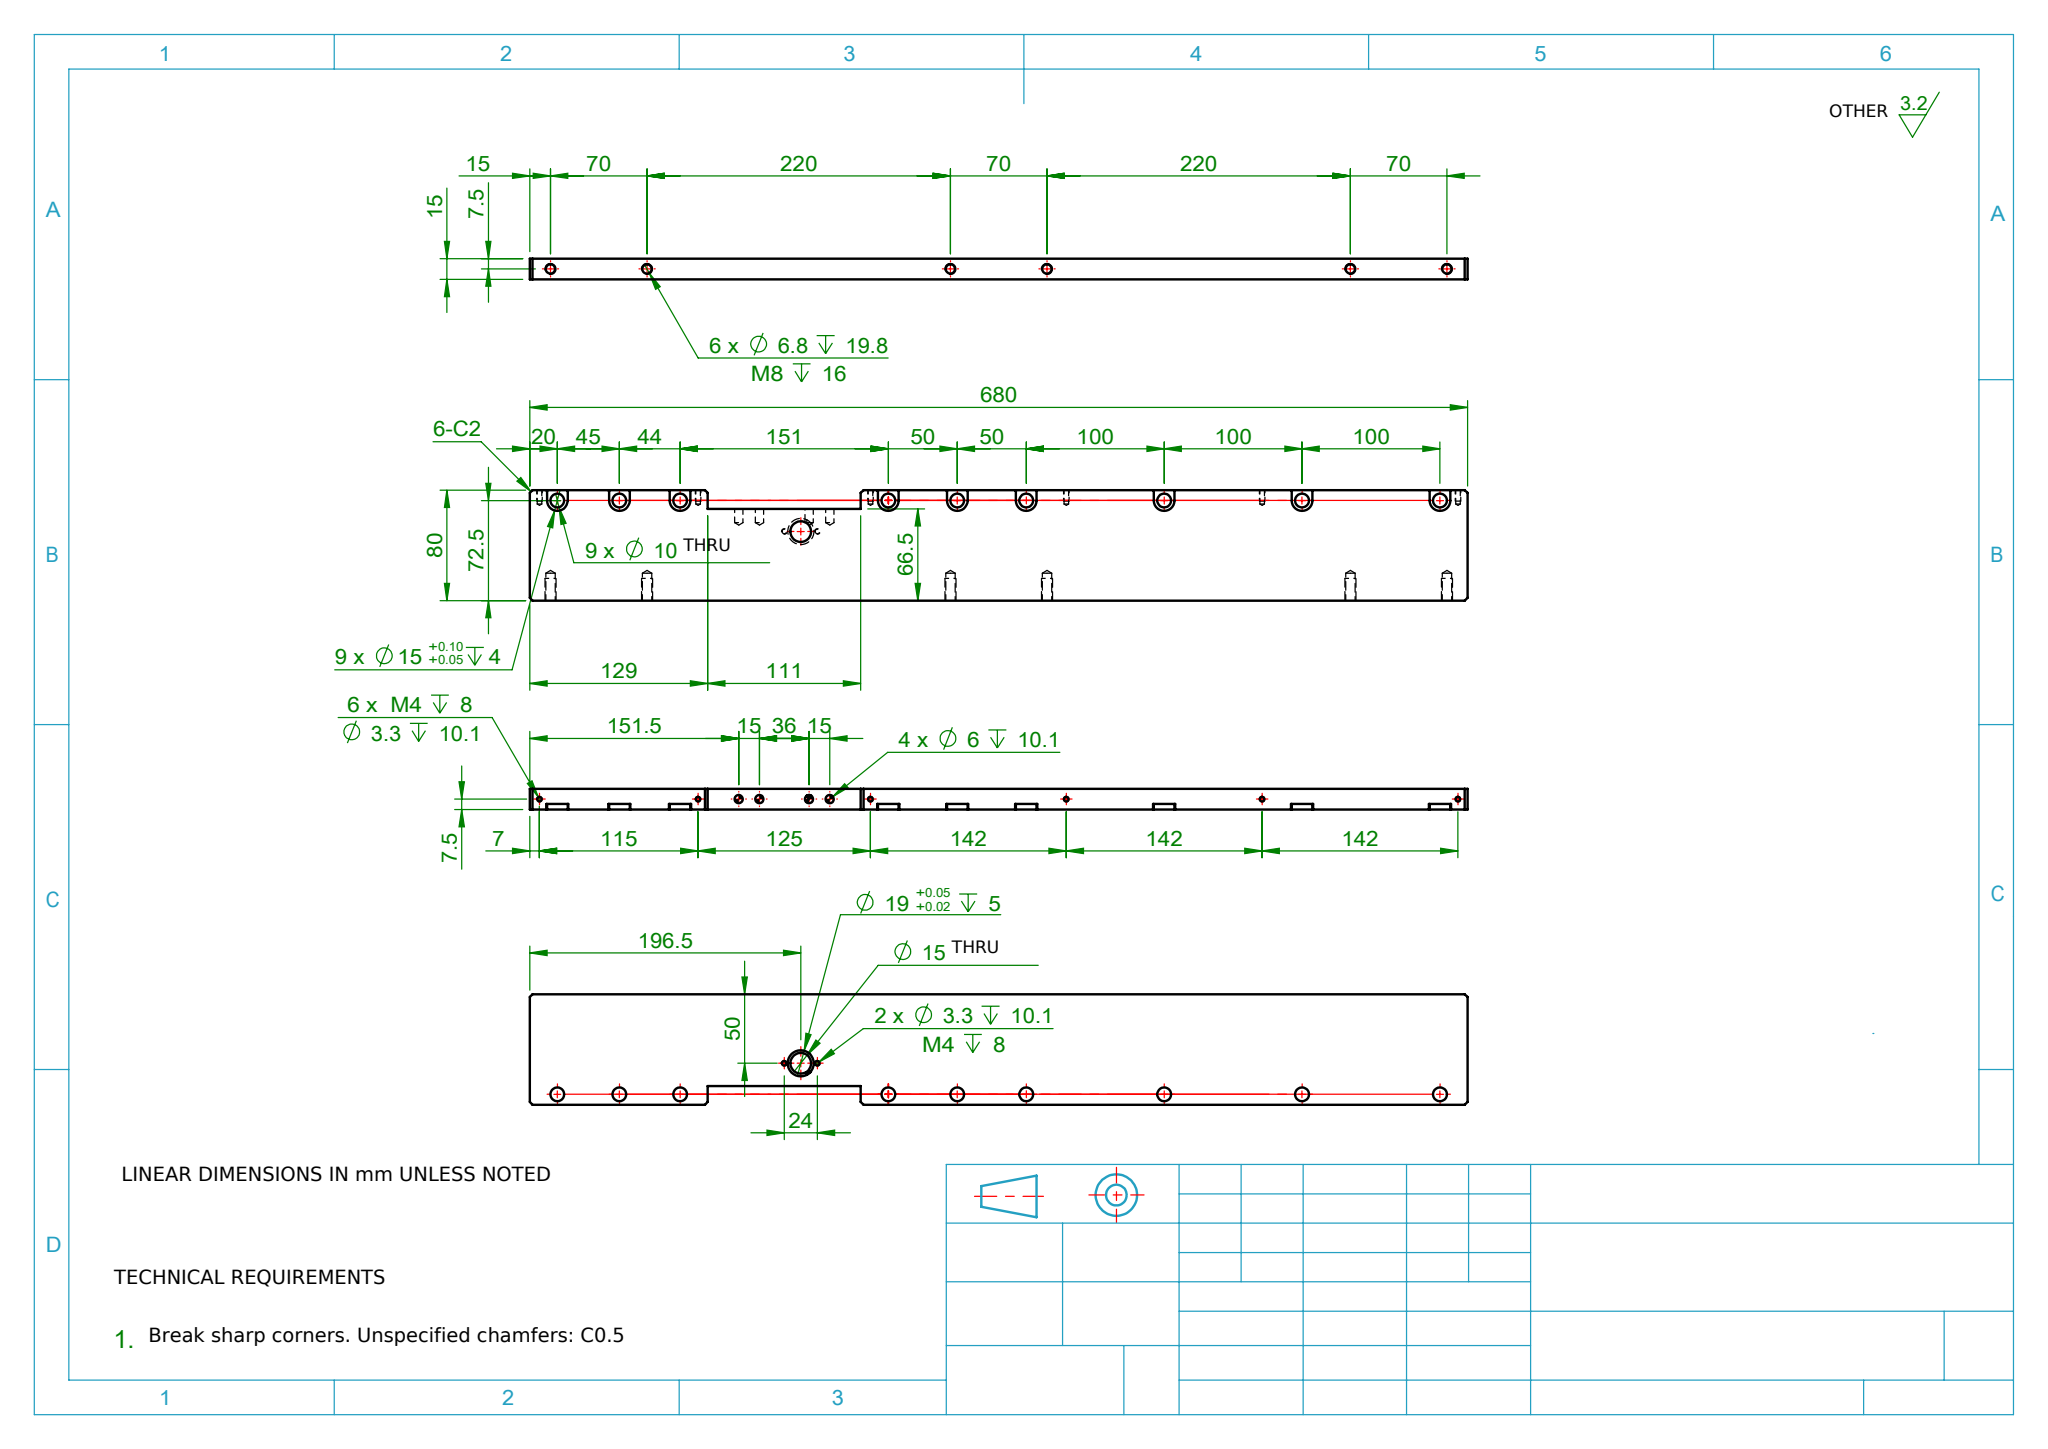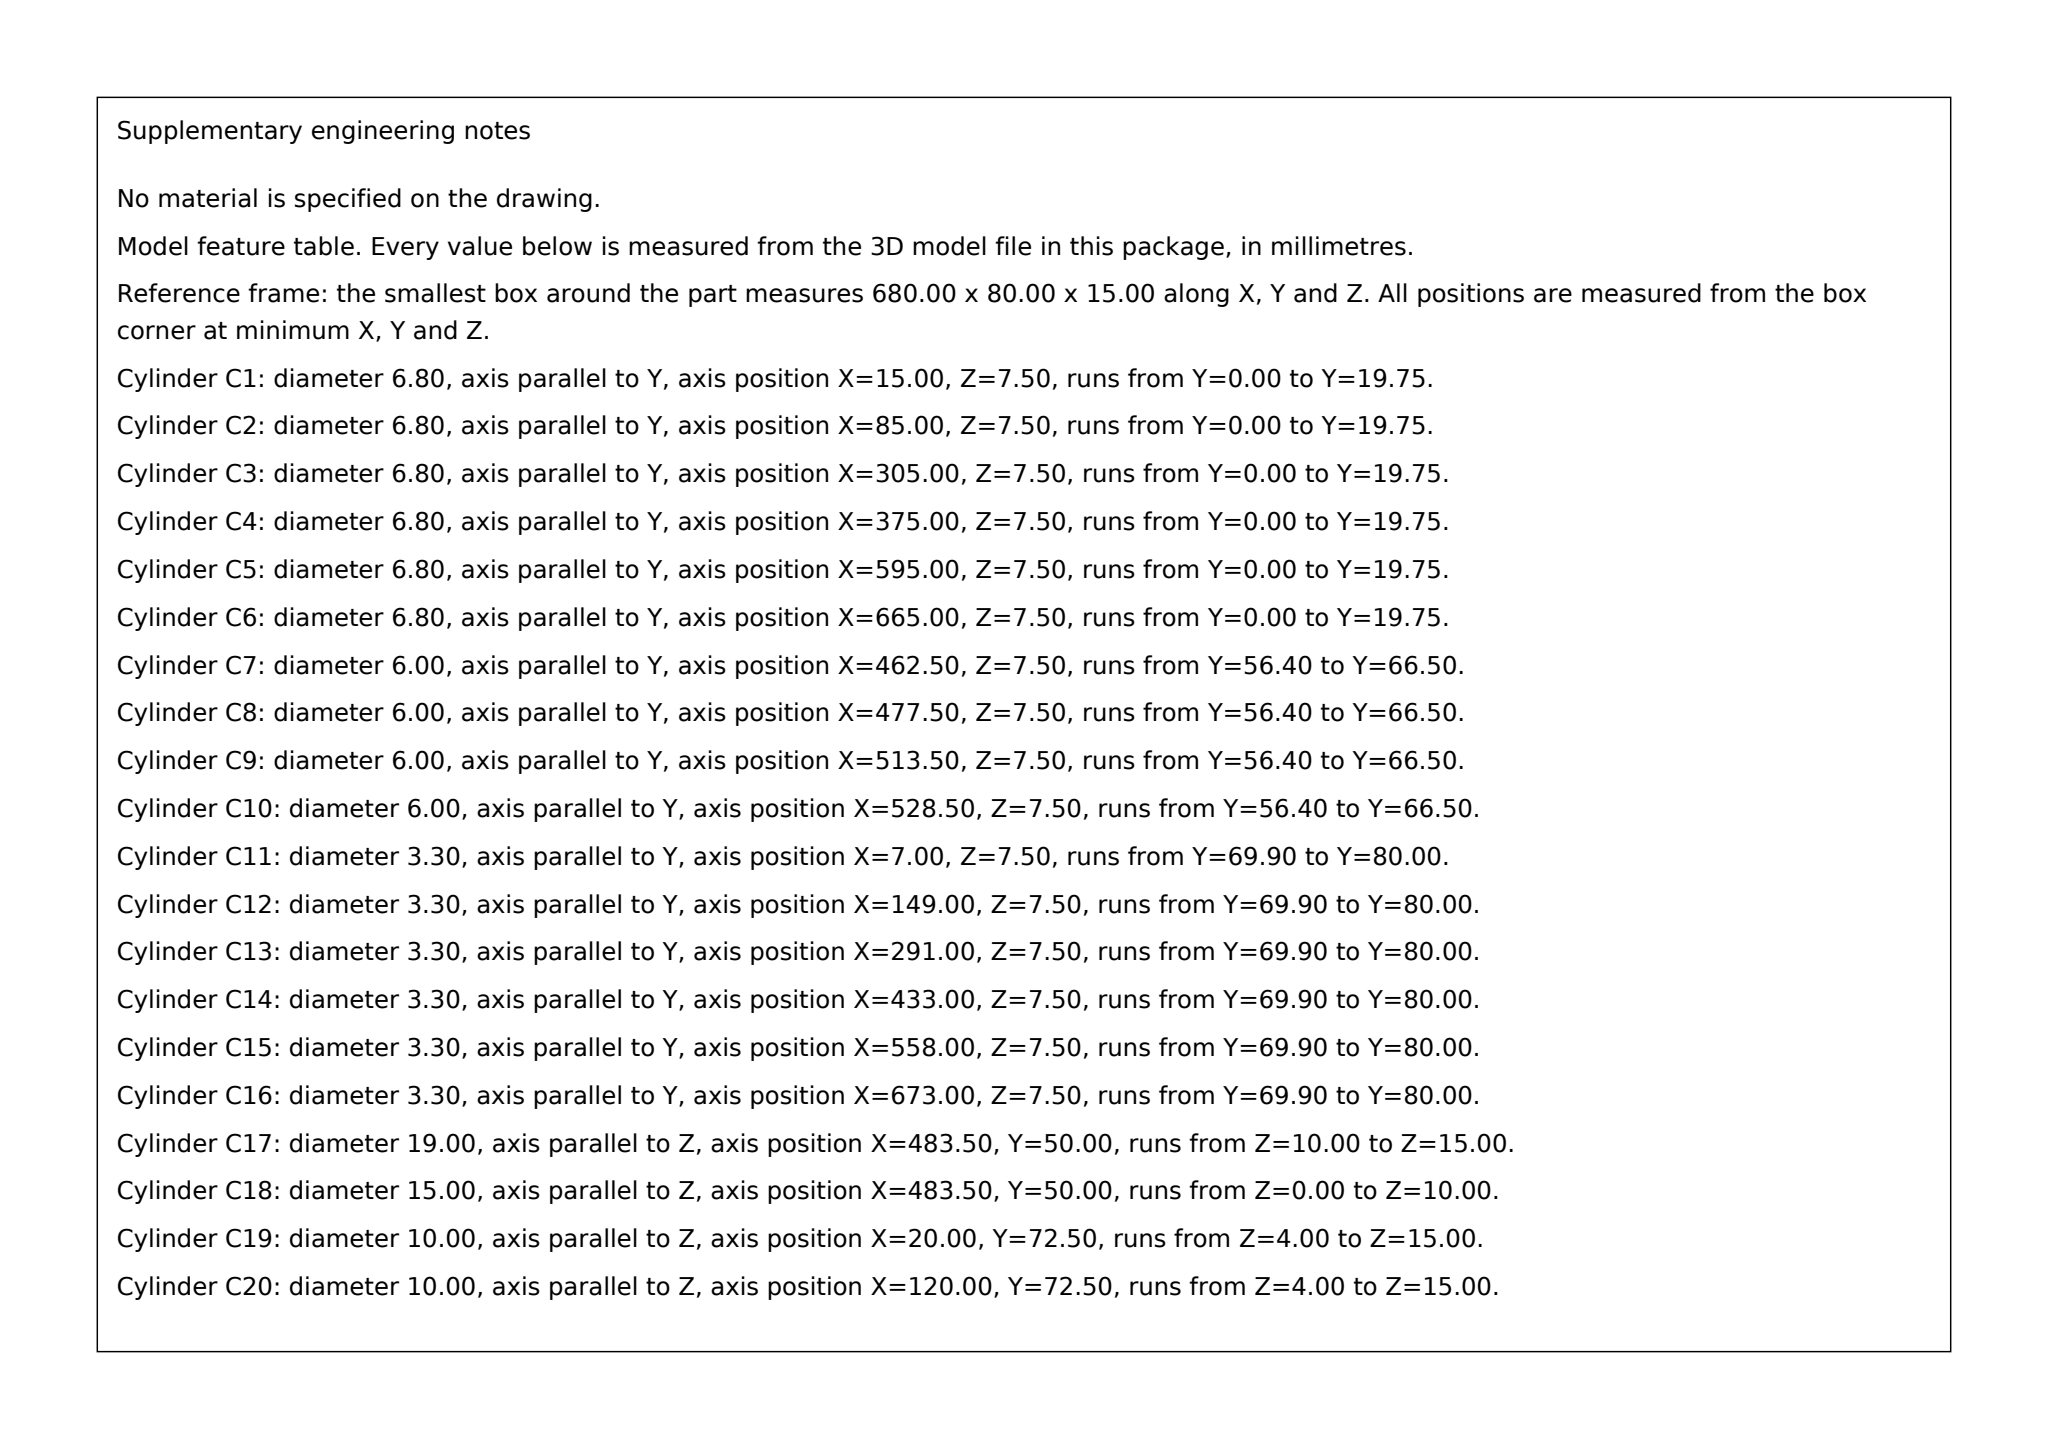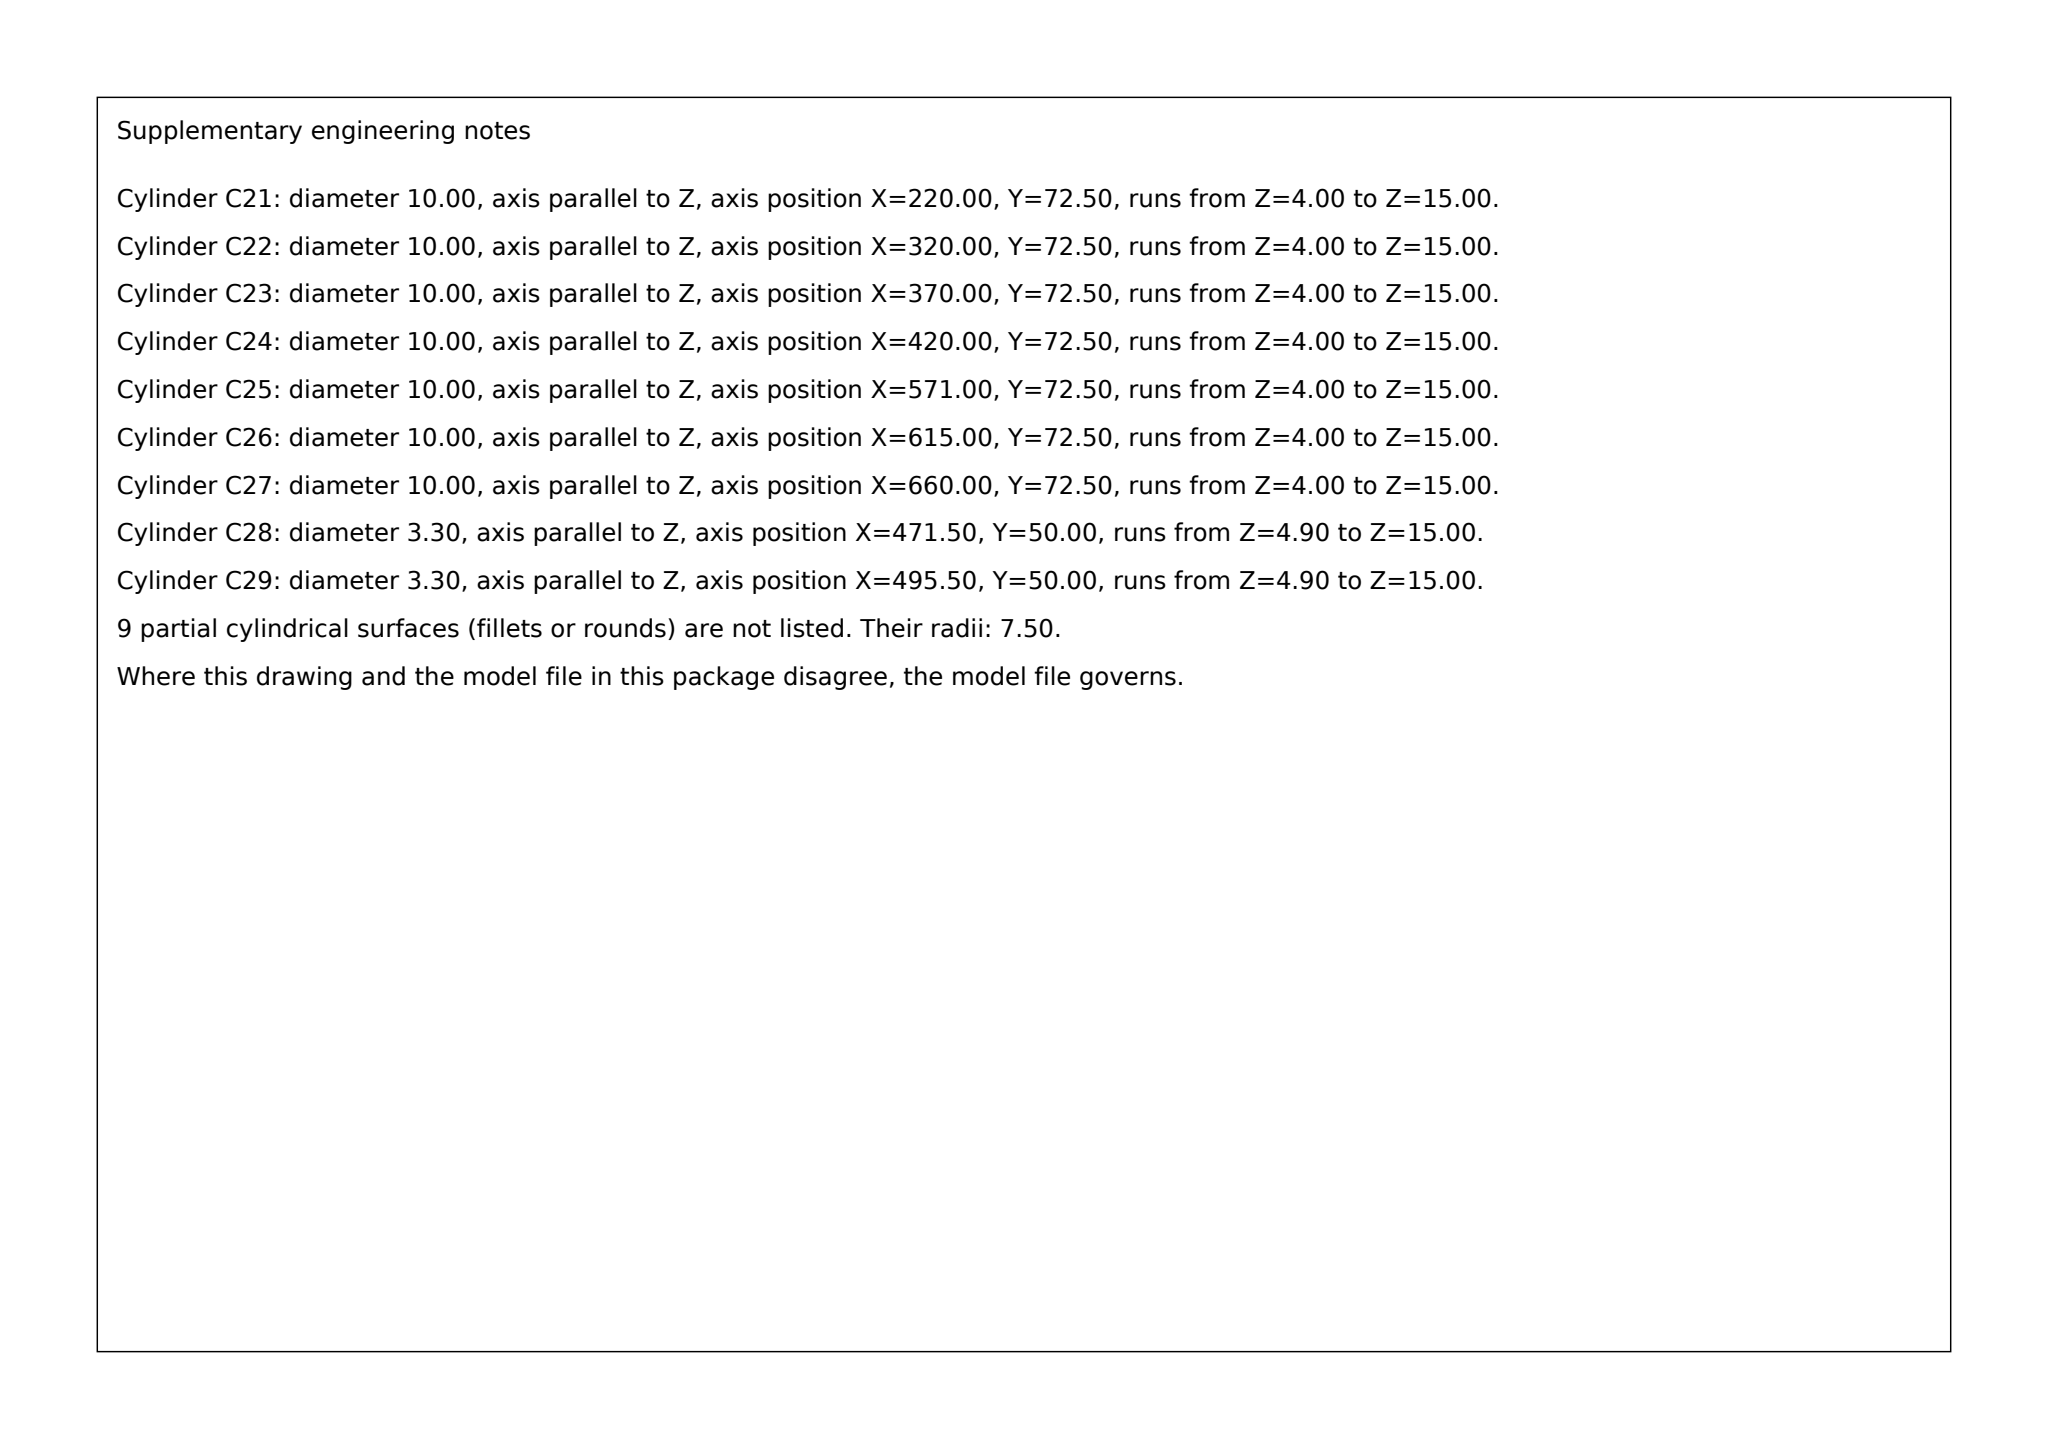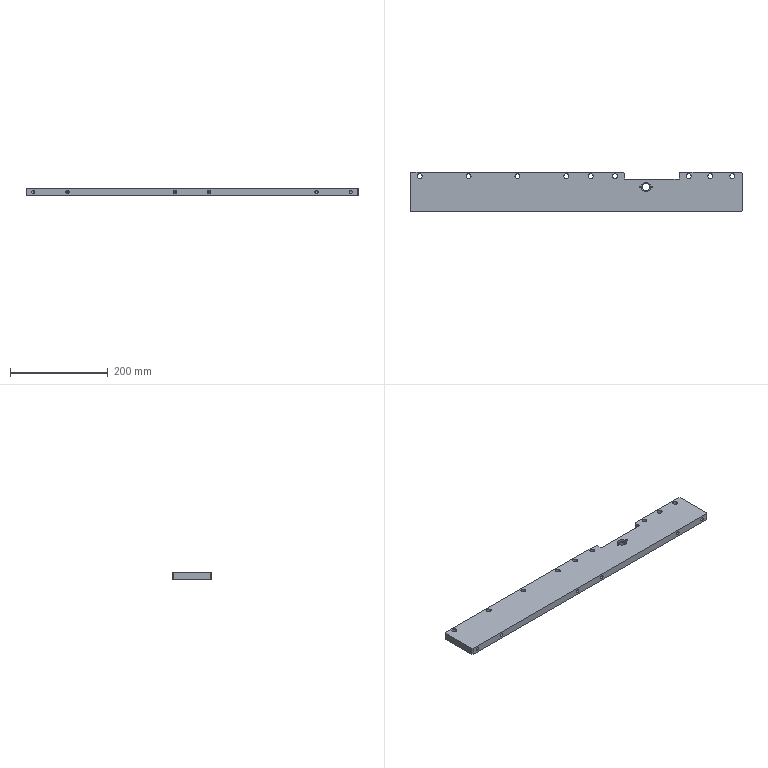Part | SolidWorks | mm | 1 solid | 165 faces | box 680 x 80 x 15 mm | volume 768770 mm3 | cylinder 67 | plane 62 | cone 36 | commonest cylinder face diameters 10 x18 3.3 x16 6.8 x12 15 x11 6 x8 19 x2
build123d program:
from build123d import *

# Parameters (mm, degrees)
SKETCH1_W                      = 440
SKETCH1_H                      = 50
BOSS_EXTRUDE1_DEPTH            = 15
HOLE_1_D                       = 10
CUT_EXTRUDE1_DEPTH             = 4
LPATTERN1_COUNT                = 3
LPATTERN1_PITCH                = 50
LPATTERN2_COUNT                = 2
LPATTERN2_PITCH                = 200
LPATTERN3_COUNT                = 2
LPATTERN3_PITCH                = 400
LPATTERN5_COUNT                = 2
LPATTERN5_PITCH                = 300
SKETCH5_W                      = 440
SKETCH5_H                      = 15
BOSS_EXTRUDE2_DEPTH            = 100
SKETCH6_W                      = 15
SKETCH6_H                      = 150
BOSS_EXTRUDE3_DEPTH            = 176
LPATTERN7_COUNT                = 2
LPATTERN7_PITCH                = 151
SKETCH7_W                      = 111
SKETCH7_H                      = 13.5
CUT_EXTRUDE2_DEPTH             = 625.244
SIZE_MM_DOWEL_PIN_HOLE_1_D     = 6
SIZE_MM_DOWEL_PIN_HOLE_1_DEPTH = 10.1
SIZE_MM_DOWEL_PIN_HOLE_1_TIP   = 1.803
SKETCH14_W                     = 15
SKETCH14_H                     = 150
BOSS_EXTRUDE4_DEPTH            = 64
LPATTERN8_COUNT                = 2
LPATTERN8_PITCH                = 195
M4_TAPPED_HOLE1_D              = 3.3
M4_TAPPED_HOLE1_DEPTH          = 10.1
M4_TAPPED_HOLE1_TIP            = 0.9914
HOLE_3_D                       = 19
HOLE_3_DEPTH                   = 5
HOLE_4_D                       = 15
SKETCH21_W                     = 680
SKETCH21_H                     = 70
CUT_EXTRUDE3_DEPTH             = 688.477
LPATTERN9_COUNT                = 2
LPATTERN9_PITCH                = 240
M8_TAPPED_HOLE1_D              = 6.8
M8_TAPPED_HOLE1_DEPTH          = 19.75
M8_TAPPED_HOLE1_TIP            = 2.043
CHAMFER1_SIZE                  = 2
CHAMFER2_SIZE                  = 0.5
M4_TAPPED_HOLE2_D              = 3.3
M4_TAPPED_HOLE2_DEPTH          = 10.1
M4_TAPPED_HOLE2_TIP            = 0.9914


with BuildPart() as part:
    # Sketch1 → Boss-Extrude1 (new body)
    with BuildSketch(Plane.XY):
        with Locations((220, 25)):
            Rectangle(SKETCH1_W, SKETCH1_H)
    extrude(amount=BOSS_EXTRUDE1_DEPTH)

    # Hole 1 (through all)
    with Locations(Plane(origin=(0, 0, 0), x_dir=(-1, 0, 0), z_dir=(0, 0, -1))):
        with Locations((-420, 42.5)):
            hole_1 = Hole(HOLE_1_D / 2)

    # Sketch4 → Cut-Extrude1 (cut)
    with BuildSketch(Plane(origin=(0, 0, 0), x_dir=(-1, 0, 0), z_dir=(0, 0, -1))):
        with BuildLine():
            Line((-427.5, 42.5), (-427.5, 50))
            Line((-427.5, 50), (-412.5, 50))
            Line((-412.5, 50), (-412.5, 42.5))
            ThreePointArc((-412.5, 42.5), (-420, 35), (-427.5, 42.5))
        make_face()
    cut_extrude1 = extrude(amount=-CUT_EXTRUDE1_DEPTH, mode=Mode.SUBTRACT)

    # LPattern1: Hole 1, Cut-Extrude1 ×3
    with Locations(*[(-i * LPATTERN1_PITCH, 0, 0) for i in range(1, LPATTERN1_COUNT)]):
        add(hole_1, mode=Mode.SUBTRACT)
        add(cut_extrude1, mode=Mode.SUBTRACT)

    # LPattern2: Hole 1, Cut-Extrude1 ×2
    with Locations(*[(-i * LPATTERN2_PITCH, 0, 0) for i in range(1, LPATTERN2_COUNT)]):
        add(hole_1, mode=Mode.SUBTRACT)
        add(cut_extrude1, mode=Mode.SUBTRACT)

    # LPattern3: Hole 1, Cut-Extrude1 ×2
    with Locations(*[(-i * LPATTERN3_PITCH, 0, 0) for i in range(1, LPATTERN3_COUNT)]):
        add(hole_1, mode=Mode.SUBTRACT)
        add(cut_extrude1, mode=Mode.SUBTRACT)

    # LPattern5: Hole 1, Cut-Extrude1 ×2
    with Locations(*[(-i * LPATTERN5_PITCH, 0, 0) for i in range(1, LPATTERN5_COUNT)]):
        add(hole_1, mode=Mode.SUBTRACT)
        add(cut_extrude1, mode=Mode.SUBTRACT)

    # Sketch5 → Boss-Extrude2 (add)
    with BuildSketch(Plane.XZ):
        with Locations((220, 7.5)):
            Rectangle(SKETCH5_W, SKETCH5_H)
    extrude(amount=BOSS_EXTRUDE2_DEPTH)

    # Sketch6 → Boss-Extrude3 (add)
    with BuildSketch(Plane(origin=(440, 0, 0), x_dir=(0, 0, -1), z_dir=(1, 0, 0))):
        with Locations((-7.5, -25)):
            Rectangle(SKETCH6_W, SKETCH6_H)
    extrude(amount=BOSS_EXTRUDE3_DEPTH)

    # LPattern7: Hole 1, Cut-Extrude1 ×2
    with Locations(*[(i * LPATTERN7_PITCH, 0, 0) for i in range(1, LPATTERN7_COUNT)]):
        add(hole_1, mode=Mode.SUBTRACT)
        add(cut_extrude1, mode=Mode.SUBTRACT)

    # Sketch7 → Cut-Extrude2 (cut, through all)
    with BuildSketch(Plane(origin=(0, 0, 0), x_dir=(-1, 0, 0), z_dir=(0, 0, -1))):
        with Locations((-495.5, 43.25)):
            Rectangle(SKETCH7_W, SKETCH7_H)
    extrude(amount=-CUT_EXTRUDE2_DEPTH, mode=Mode.SUBTRACT)

    # Size mm Dowel Pin Hole 1
    with Locations(Plane(origin=(0, 36.5, 0), x_dir=(1, 0, 0), z_dir=(0, 1, 0))):
        with Locations((528.5, -7.5), (513.5, -7.5), (477.5, -7.5), (462.5, -7.5)):
            Hole(SIZE_MM_DOWEL_PIN_HOLE_1_D / 2, depth=SIZE_MM_DOWEL_PIN_HOLE_1_DEPTH)
            with Locations((0, 0, -(SIZE_MM_DOWEL_PIN_HOLE_1_DEPTH + SIZE_MM_DOWEL_PIN_HOLE_1_TIP / 2))):  # 118° drill point
                Cone(0, SIZE_MM_DOWEL_PIN_HOLE_1_D / 2, SIZE_MM_DOWEL_PIN_HOLE_1_TIP, mode=Mode.SUBTRACT)

    # Sketch14 → Boss-Extrude4 (add)
    with BuildSketch(Plane(origin=(616, 0, 0), x_dir=(0, 0, -1), z_dir=(1, 0, 0))):
        with Locations((-7.5, -25)):
            Rectangle(SKETCH14_W, SKETCH14_H)
    extrude(amount=BOSS_EXTRUDE4_DEPTH)

    # LPattern8: Hole 1, Cut-Extrude1 ×2
    with Locations(*[(i * LPATTERN8_PITCH, 0, 0) for i in range(1, LPATTERN8_COUNT)]):
        add(hole_1, mode=Mode.SUBTRACT)
        add(cut_extrude1, mode=Mode.SUBTRACT)

    # M4 Tapped Hole1
    with Locations(Plane(origin=(0, 50, 0), x_dir=(1, 0, 0), z_dir=(0, 1, 0))):
        with Locations((291, -7.5), (149, -7.5), (7, -7.5), (673, -7.5), (558, -7.5), (433, -7.5)):
            Hole(M4_TAPPED_HOLE1_D / 2, depth=M4_TAPPED_HOLE1_DEPTH)
            with Locations((0, 0, -(M4_TAPPED_HOLE1_DEPTH + M4_TAPPED_HOLE1_TIP / 2))):  # 118° drill point
                Cone(0, M4_TAPPED_HOLE1_D / 2, M4_TAPPED_HOLE1_TIP, mode=Mode.SUBTRACT)

    # Hole 3
    with Locations(Plane.XY.offset(15)):
        with Locations((483.5, 20)):
            Hole(HOLE_3_D / 2, depth=HOLE_3_DEPTH)

    # Hole 4 (through all)
    with Locations(Plane.XY.offset(10)):
        with Locations((483.5, 20)):
            Hole(HOLE_4_D / 2)

    # Sketch21 → Cut-Extrude3 (cut, through all)
    with BuildSketch(Plane.XY.offset(15)):
        with Locations((340, -65)):
            Rectangle(SKETCH21_W, SKETCH21_H)
    extrude(amount=-CUT_EXTRUDE3_DEPTH, mode=Mode.SUBTRACT)

    # LPattern9: Hole 1, Cut-Extrude1 ×2
    with Locations(*[(i * LPATTERN9_PITCH, 0, 0) for i in range(1, LPATTERN9_COUNT)]):
        add(hole_1, mode=Mode.SUBTRACT)
        add(cut_extrude1, mode=Mode.SUBTRACT)

    # M8 Tapped Hole1
    with Locations(Plane(origin=(0, -30, 0), x_dir=(-1, 0, 0), z_dir=(0, -1, 0))):
        with Locations((-665, -7.5), (-595, -7.5), (-375, -7.5), (-305, -7.5), (-85, -7.5), (-15, -7.5)):
            Hole(M8_TAPPED_HOLE1_D / 2, depth=M8_TAPPED_HOLE1_DEPTH)
            with Locations((0, 0, -(M8_TAPPED_HOLE1_DEPTH + M8_TAPPED_HOLE1_TIP / 2))):  # 118° drill point
                Cone(0, M8_TAPPED_HOLE1_D / 2, M8_TAPPED_HOLE1_TIP, mode=Mode.SUBTRACT)

    # Chamfer1
    chamfer1_edges = [part.edges().sort_by_distance(p)[0] for p in [
        (551, 50, 7.5),
        (440, 50, 7.5),
        (680, 50, 7.5),
        (680, -30, 7.5),
        (0, -30, 7.5),
        (0, 50, 7.5),
    ]]
    chamfer(chamfer1_edges, length=CHAMFER1_SIZE)

    # Chamfer2
    chamfer2_edges = [part.edges().sort_by_distance(p)[0] for p in [
        (27.5, 50, 2),
        (12.5, 50, 2),
        (127.5, 50, 2),
        (112.5, 50, 2),
        (578.5, 50, 2),
        (563.5, 50, 2),
        (622.5, 50, 2),
        (607.5, 50, 2),
        (427.5, 50, 2),
        (412.5, 50, 2),
        (667.5, 50, 2),
        (652.5, 50, 2),
        (377.5, 50, 2),
        (362.5, 50, 2),
        (327.5, 50, 2),
        (312.5, 50, 2),
        (227.5, 50, 2),
        (212.5, 50, 2),
    ]]
    chamfer(chamfer2_edges, length=CHAMFER2_SIZE)

    # M4 Tapped Hole2
    with Locations(Plane.XY.offset(15)):
        with Locations((471.5, 20), (495.5, 20)):
            Hole(M4_TAPPED_HOLE2_D / 2, depth=M4_TAPPED_HOLE2_DEPTH)
            with Locations((0, 0, -(M4_TAPPED_HOLE2_DEPTH + M4_TAPPED_HOLE2_TIP / 2))):  # 118° drill point
                Cone(0, M4_TAPPED_HOLE2_D / 2, M4_TAPPED_HOLE2_TIP, mode=Mode.SUBTRACT)


solid = part.part